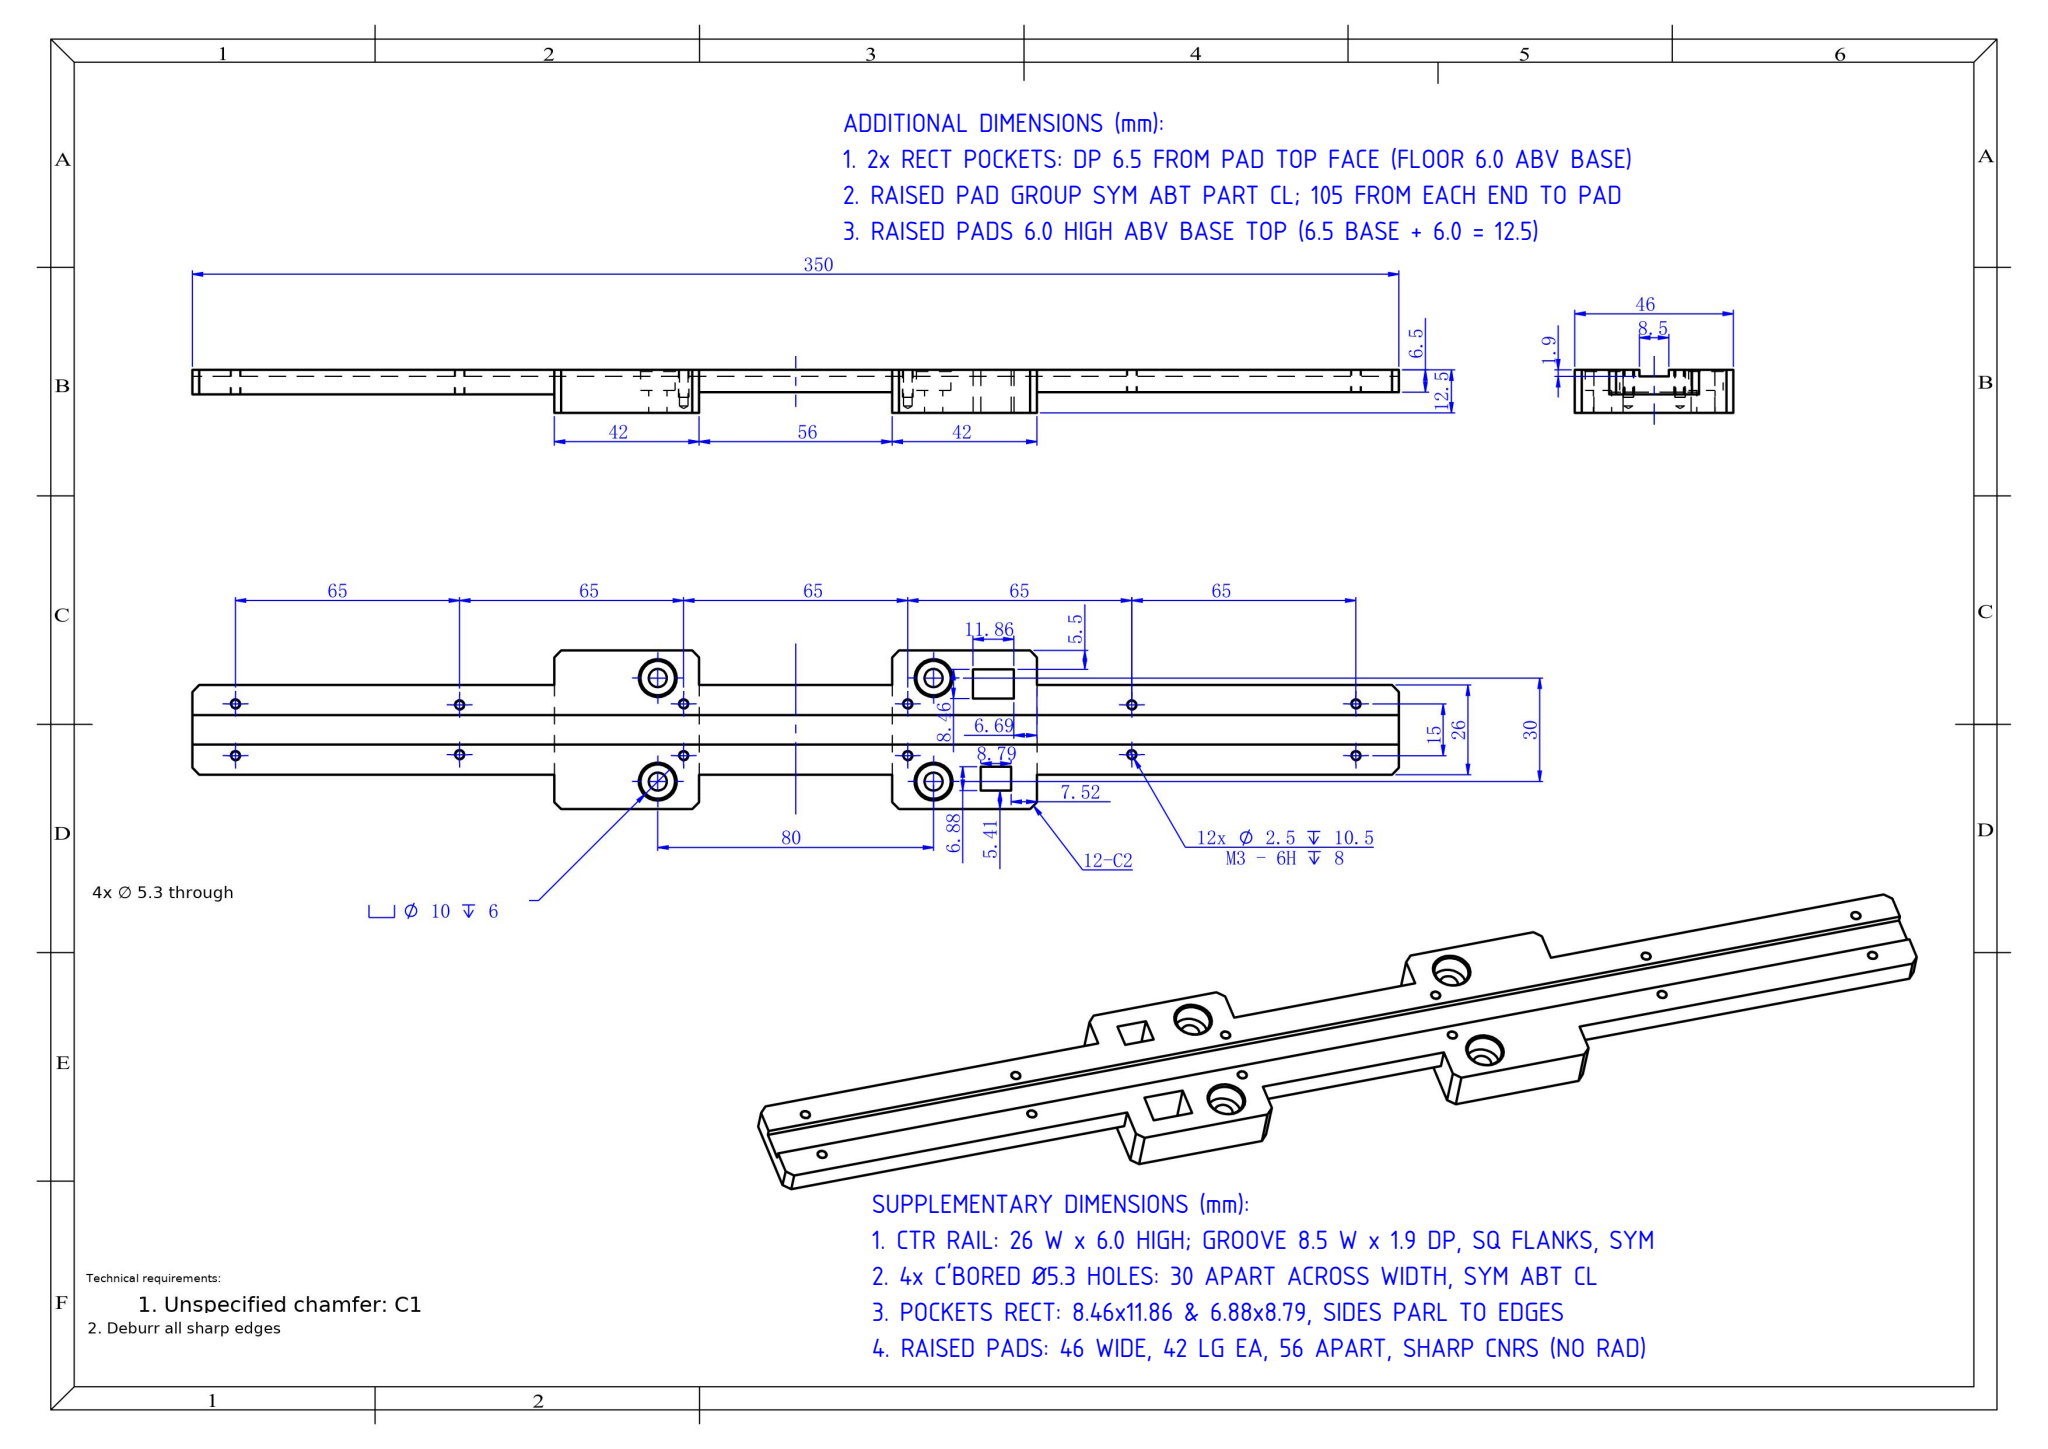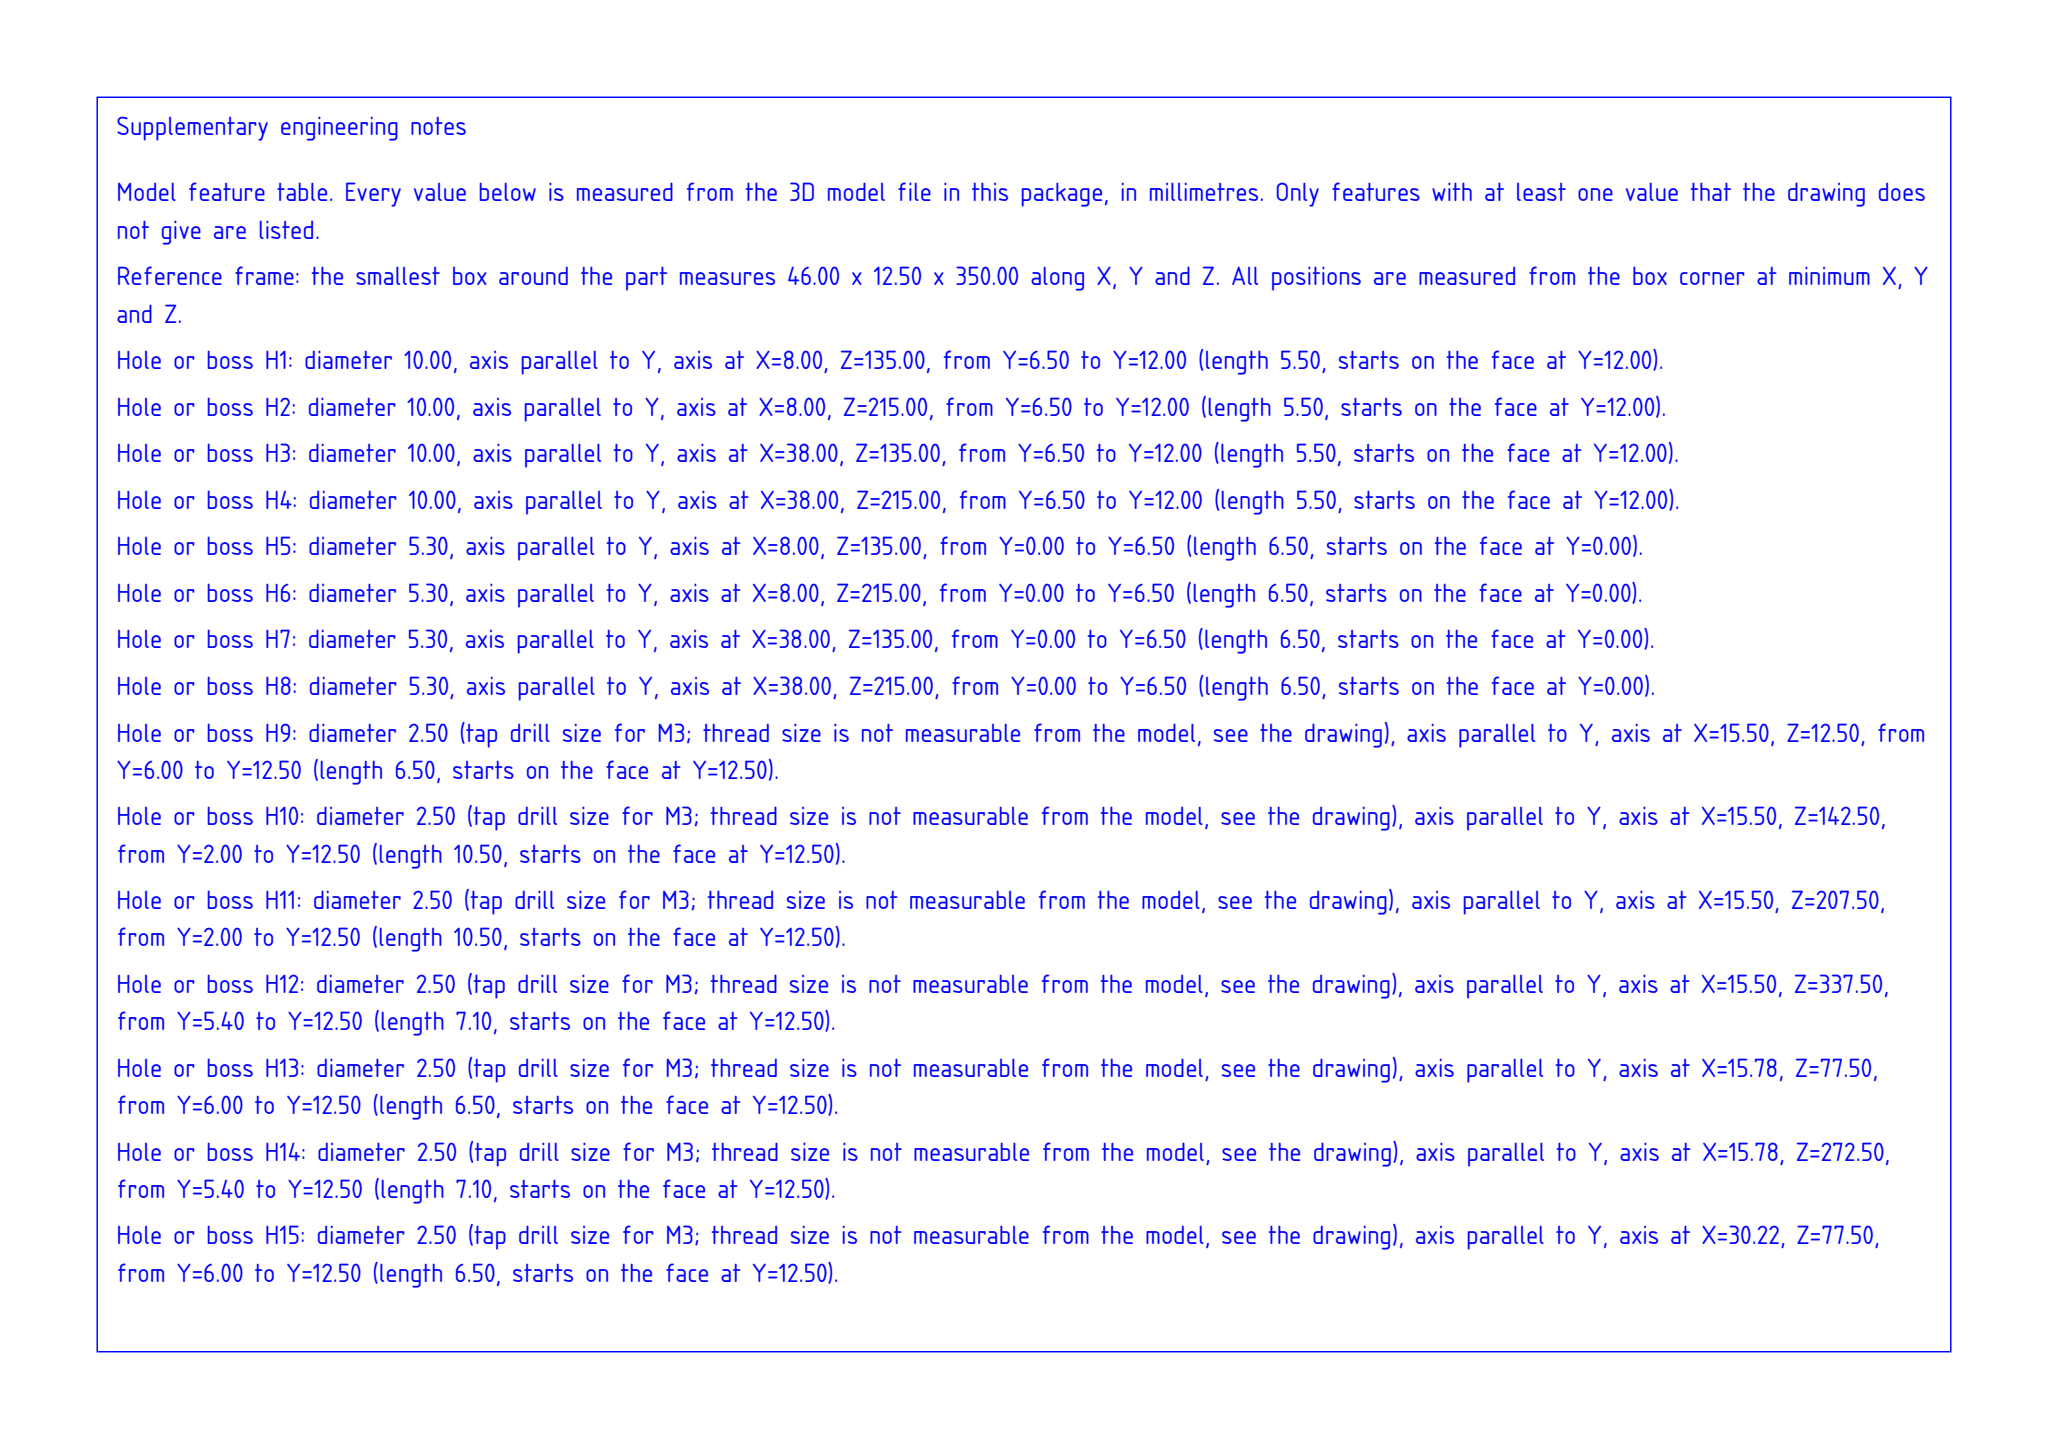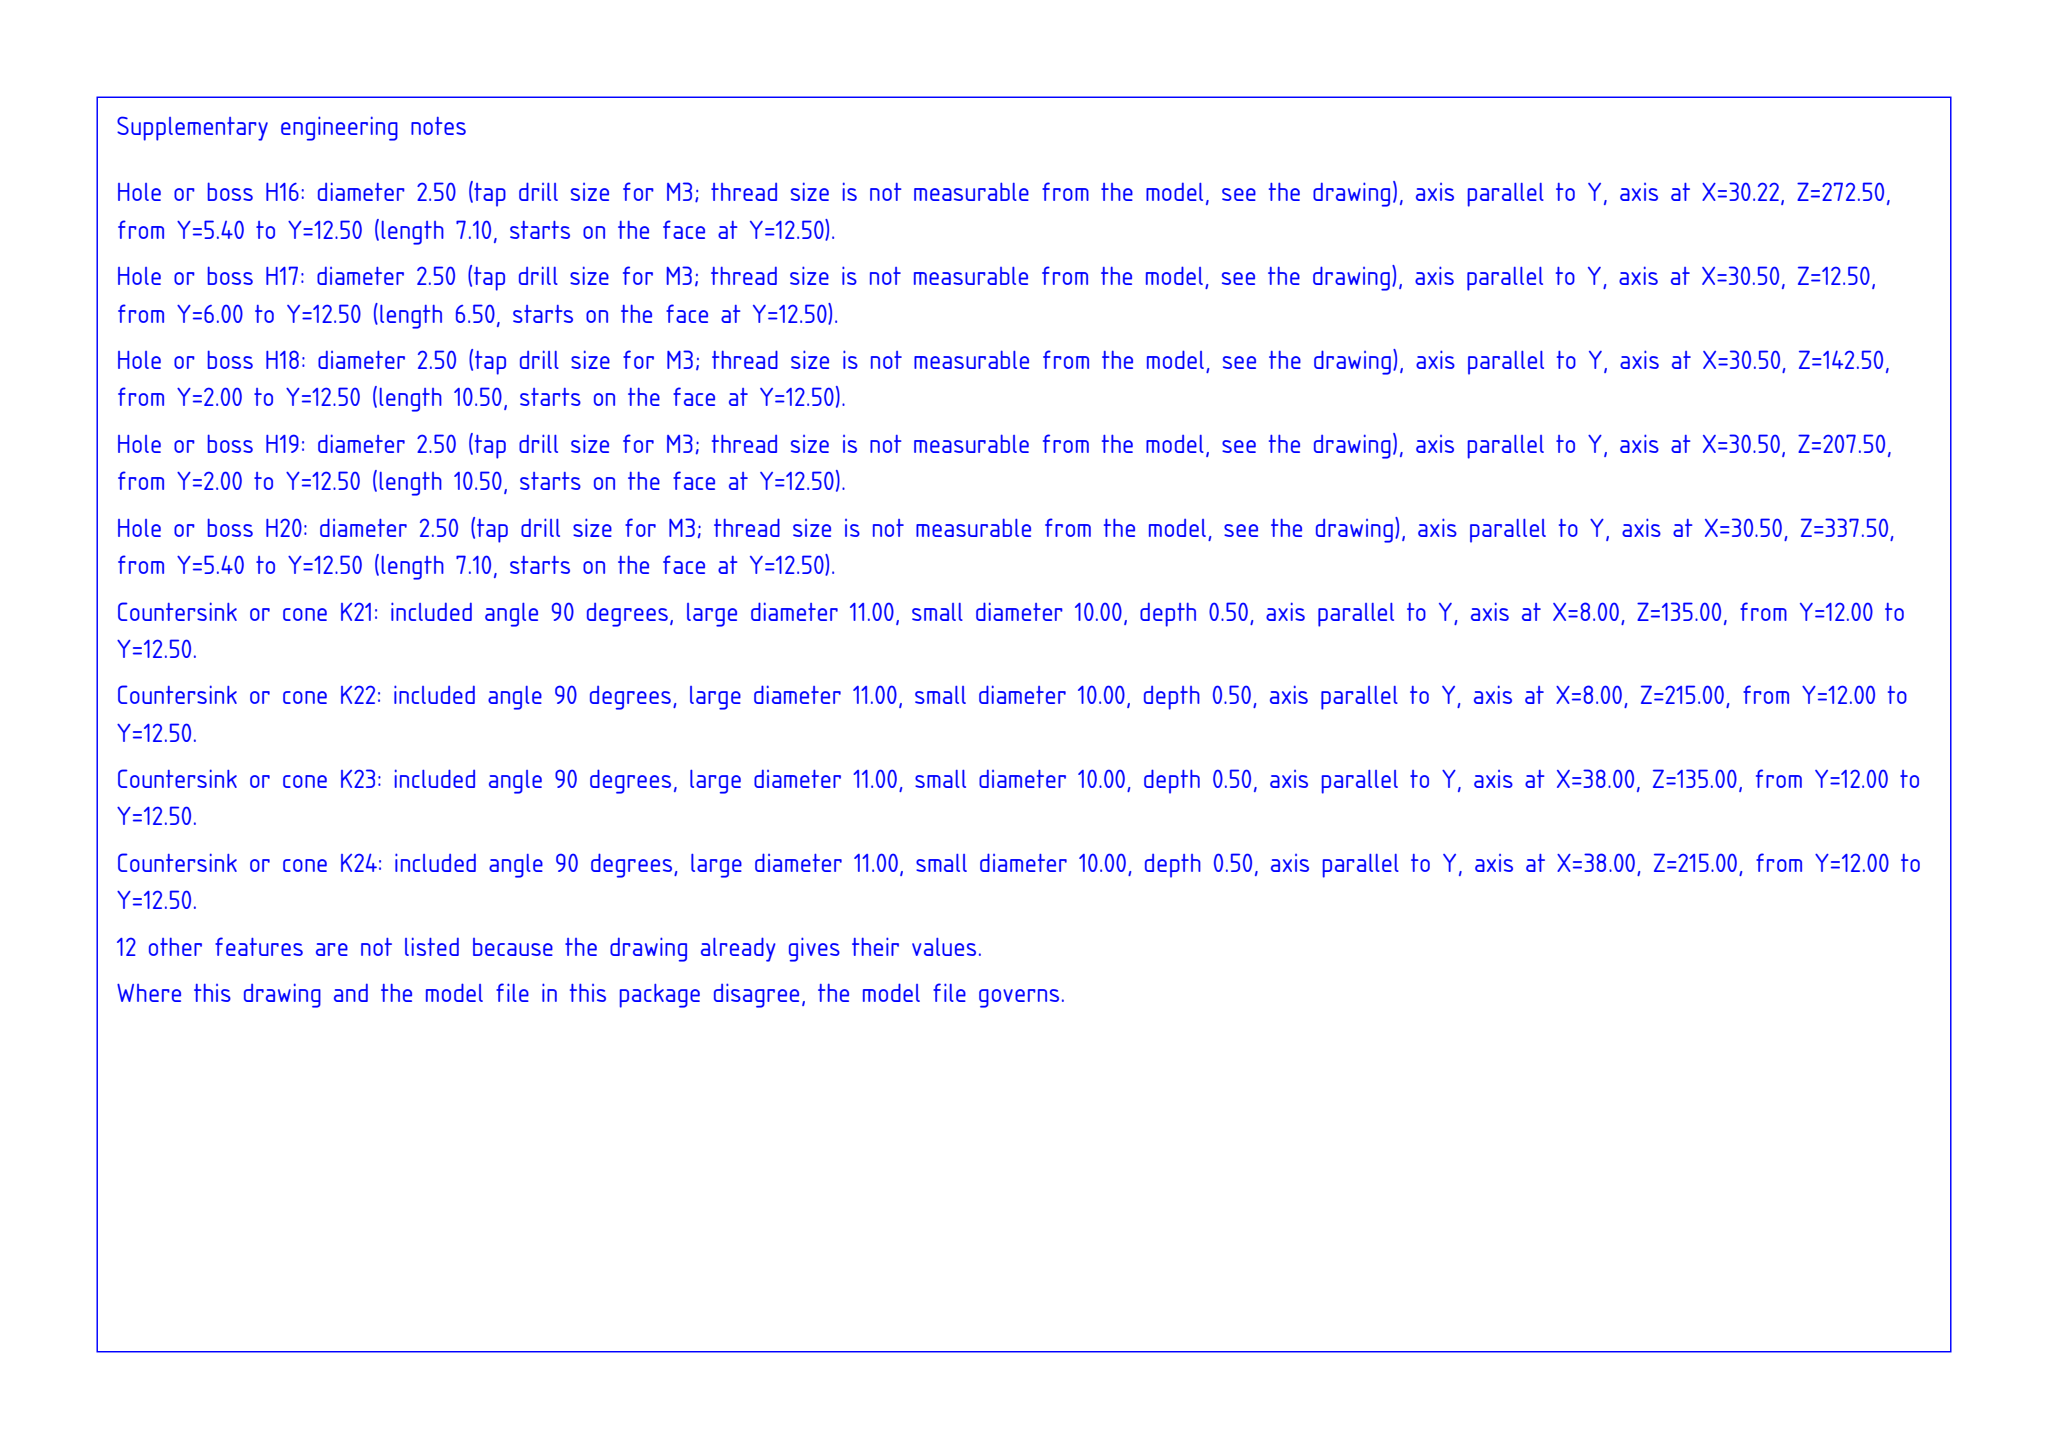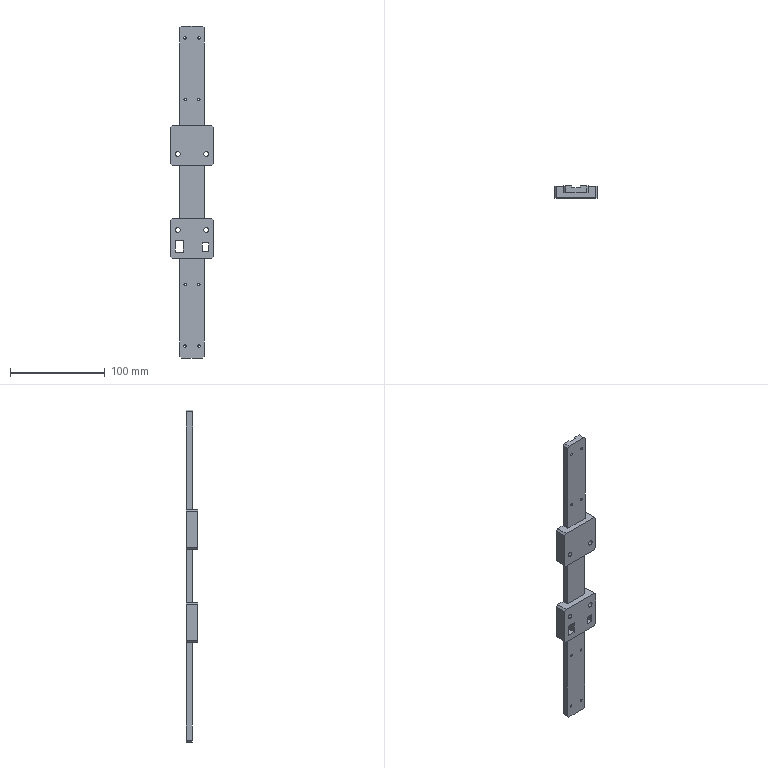Part | SolidWorks | mm | 1 solid | 106 faces | box 46 x 12.5 x 350 mm | volume 84021 mm3 | plane 50 | cylinder 40 | cone 16 | commonest cylinder face diameters 2.5 x24 10 x8 5.3 x8
build123d program:
from build123d import *

# Parameters (mm, degrees)
BOSS_EXTRUDE1_DEPTH                             = 350
M5_HEX_SOCKET_HEAD_CAP_SCREW_CBORE1_D           = 5.3
M5_HEX_SOCKET_HEAD_CAP_SCREW_CBORE1_CBORE_D     = 10
M5_HEX_SOCKET_HEAD_CAP_SCREW_CBORE1_CBORE_DEPTH = 6
CHAMFER1_SIZE                                   = 0.5
SKETCH7_W                                       = 10
SKETCH7_H                                       = 105
CUT_EXTRUDE3_DEPTH                              = 366.908
CHAMFER2_SIZE                                   = 2
SKETCH10_W                                      = 10
SKETCH10_H                                      = 56
CUT_EXTRUDE4_DEPTH                              = 366.908
CHAMFER3_SIZE                                   = 2
SKETCH11_W                                      = 105
SKETCH11_H                                      = 6
SKETCH11_W_2                                    = 56
CUT_EXTRUDE5_DEPTH                              = 355.582
M3_TAPPED_HOLE1_AT_2_COUNT                      = 2
M3_TAPPED_HOLE1_AT_2_PITCH                      = 65.001
M3_TAPPED_HOLE1_AT_3_COUNT                      = 2
M3_TAPPED_HOLE1_AT_3_PITCH                      = 130
M3_TAPPED_HOLE1_AT_4_COUNT                      = 2
M3_TAPPED_HOLE1_AT_4_PITCH                      = 195
M3_TAPPED_HOLE1_AT_5_COUNT                      = 2
M3_TAPPED_HOLE1_AT_5_PITCH                      = 260
M3_TAPPED_HOLE1_AT_6_COUNT                      = 2
M3_TAPPED_HOLE1_AT_6_PITCH                      = 325
SKETCH14_W                                      = 6.885
SKETCH14_H                                      = 8.792
SKETCH14_W_2                                    = 8.461
SKETCH14_H_2                                    = 11.861
CUT_EXTRUDE6_DEPTH                              = 38


with BuildPart() as part:
    # Sketch1 → Boss-Extrude1 (new body)
    with BuildSketch(Plane.XY):
        Polygon((-105.984, 43.956), (-87.234, 43.956), (-87.234, 42.056), (-78.734, 42.056), (-78.734, 43.956), (-59.984, 43.956), (-59.984, 31.456), (-105.984, 31.456), align=None)
    extrude(amount=BOSS_EXTRUDE1_DEPTH)

    # M5 Hex Socket Head Cap Screw CBORE1 (through all)
    with Locations(Plane(origin=(0, 43.956, 0), x_dir=(1, 0, 0), z_dir=(0, 1, 0))):
        with Locations((-67.984, -135), (-67.984, -215), (-97.984, -135), (-97.984, -215)):
            CounterBoreHole(M5_HEX_SOCKET_HEAD_CAP_SCREW_CBORE1_D / 2, M5_HEX_SOCKET_HEAD_CAP_SCREW_CBORE1_CBORE_D / 2, M5_HEX_SOCKET_HEAD_CAP_SCREW_CBORE1_CBORE_DEPTH)

    # Chamfer1
    chamfer1_edges = [part.edges().sort_by_distance(p)[0] for p in [
        (-102.984, 43.956, 215),
        (-102.984, 43.956, 135),
        (-72.984, 43.956, 215),
        (-72.984, 43.956, 135),
    ]]
    chamfer(chamfer1_edges, length=CHAMFER1_SIZE)

    # Sketch7 → Cut-Extrude3 (cut, through all)
    with BuildSketch(Plane(origin=(0, 43.956, 0), x_dir=(1, 0, 0), z_dir=(0, 1, 0))):
        with Locations((-100.984, -52.5)):
            Rectangle(SKETCH7_W, SKETCH7_H)
        with Locations((-100.984, -297.5)):
            Rectangle(SKETCH7_W, SKETCH7_H)
        with Locations((-64.984, -297.5)):
            Rectangle(SKETCH7_W, SKETCH7_H)
        with Locations((-64.984, -52.5)):
            Rectangle(SKETCH7_W, SKETCH7_H)
    extrude(amount=-CUT_EXTRUDE3_DEPTH, mode=Mode.SUBTRACT)

    # Chamfer2
    chamfer2_edges = [part.edges().sort_by_distance(p)[0] for p in [
        (-69.984, 37.706, 0),
        (-59.984, 37.706, 105),
        (-95.984, 37.706, 0),
        (-105.984, 37.706, 105),
        (-105.984, 37.706, 245),
        (-95.984, 37.706, 350),
        (-69.984, 37.706, 350),
        (-59.984, 37.706, 245),
    ]]
    chamfer(chamfer2_edges, length=CHAMFER2_SIZE)

    # Sketch10 → Cut-Extrude4 (cut, through all)
    with BuildSketch(Plane(origin=(0, 43.956, 0), x_dir=(1, 0, 0), z_dir=(0, 1, 0))):
        with Locations((-64.984, -175)):
            Rectangle(SKETCH10_W, SKETCH10_H)
        with Locations((-100.984, -175)):
            Rectangle(SKETCH10_W, SKETCH10_H)
    extrude(amount=-CUT_EXTRUDE4_DEPTH, mode=Mode.SUBTRACT)

    # Chamfer3
    chamfer3_edges = [part.edges().sort_by_distance(p)[0] for p in [
        (-59.984, 37.706, 147),
        (-59.984, 37.706, 203),
        (-105.984, 37.706, 203),
        (-105.984, 37.706, 147),
    ]]
    chamfer(chamfer3_edges, length=CHAMFER3_SIZE)

    # Sketch11 → Cut-Extrude5 (cut, through all)
    with BuildSketch(Plane.ZY.offset(95.984)):
        with Locations((52.5, 34.456)):
            Rectangle(SKETCH11_W, SKETCH11_H)
        with Locations((175, 34.456)):
            Rectangle(SKETCH11_W_2, SKETCH11_H)
        with Locations((297.5, 33.856)):
            Rectangle(SKETCH11_W, SKETCH11_H)
    extrude(amount=-CUT_EXTRUDE5_DEPTH, mode=Mode.SUBTRACT)

    # Sketch13 → M3 Tapped Hole1 (revolve, cut)
    with BuildSketch(Plane(origin=(-90.484, 43.956, 337.5), x_dir=(0, 0, 1), z_dir=(1, 0, 0))):
        Polygon((0, 0), (0, 11.251), (1.25, 10.5), (1.25, 0), align=None)
    m3_tapped_hole1 = revolve(axis=Axis((-90.484, 50.306, 337.5), (0, -1, 0)), mode=Mode.SUBTRACT)

    # M3 Tapped Hole1 at 2: M3 Tapped Hole1 ×2
    with Locations(*[Vector(0.004316, 0, -1) * (i * M3_TAPPED_HOLE1_AT_2_PITCH) for i in range(1, M3_TAPPED_HOLE1_AT_2_COUNT)]):
        add(m3_tapped_hole1, mode=Mode.SUBTRACT)

    # M3 Tapped Hole1 at 3: M3 Tapped Hole1 ×2
    with Locations(*[(0, 0, -i * M3_TAPPED_HOLE1_AT_3_PITCH) for i in range(1, M3_TAPPED_HOLE1_AT_3_COUNT)]):
        add(m3_tapped_hole1, mode=Mode.SUBTRACT)

    # M3 Tapped Hole1 at 4: M3 Tapped Hole1 ×2
    with Locations(*[(0, 0, -i * M3_TAPPED_HOLE1_AT_4_PITCH) for i in range(1, M3_TAPPED_HOLE1_AT_4_COUNT)]):
        add(m3_tapped_hole1, mode=Mode.SUBTRACT)

    # M3 Tapped Hole1 at 5: M3 Tapped Hole1 ×2
    with Locations(*[Vector(0.001079, 0, -1) * (i * M3_TAPPED_HOLE1_AT_5_PITCH) for i in range(1, M3_TAPPED_HOLE1_AT_5_COUNT)]):
        add(m3_tapped_hole1, mode=Mode.SUBTRACT)

    # M3 Tapped Hole1 at 6: M3 Tapped Hole1 ×2
    with Locations(*[(0, 0, -i * M3_TAPPED_HOLE1_AT_6_PITCH) for i in range(1, M3_TAPPED_HOLE1_AT_6_COUNT)]):
        add(m3_tapped_hole1, mode=Mode.SUBTRACT)

    # Mirror1: M3 Tapped Hole1 across plane
    add(m3_tapped_hole1.mirror(Plane(origin=(-82.984, 0, 0), x_dir=(0, 0, 1), z_dir=(1, 0, 0))), mode=Mode.SUBTRACT)

    # Mirror1 copy 1 sketch → Mirror1 copy 1 (revolve, cut)
    with BuildSketch(Plane(origin=(-75.764, 43.956, 272.5), x_dir=(0, 0, 1), z_dir=(-1, 0, 0))):
        Polygon((0, 0), (0, -11.251), (1.25, -10.5), (1.25, 0), align=None)
    revolve(axis=Axis((-75.764, 50.306, 272.5), (0, 1, 0)), mode=Mode.SUBTRACT)

    # Mirror1 copy 2 sketch → Mirror1 copy 2 (revolve, cut)
    with BuildSketch(Plane(origin=(-75.484, 43.956, 207.5), x_dir=(0, 0, 1), z_dir=(-1, 0, 0))):
        Polygon((0, 0), (0, -11.251), (1.25, -10.5), (1.25, 0), align=None)
    revolve(axis=Axis((-75.484, 50.306, 207.5), (0, 1, 0)), mode=Mode.SUBTRACT)

    # Mirror1 copy 3 sketch → Mirror1 copy 3 (revolve, cut)
    with BuildSketch(Plane(origin=(-75.484, 43.956, 142.5), x_dir=(0, 0, 1), z_dir=(-1, 0, 0))):
        Polygon((0, 0), (0, -11.251), (1.25, -10.5), (1.25, 0), align=None)
    revolve(axis=Axis((-75.484, 50.306, 142.5), (0, 1, 0)), mode=Mode.SUBTRACT)

    # Mirror1 copy 4 sketch → Mirror1 copy 4 (revolve, cut)
    with BuildSketch(Plane(origin=(-75.764, 43.956, 77.5), x_dir=(0, 0, 1), z_dir=(-1, 0, 0))):
        Polygon((0, 0), (0, -11.251), (1.25, -10.5), (1.25, 0), align=None)
    revolve(axis=Axis((-75.764, 50.306, 77.5), (0, 1, 0)), mode=Mode.SUBTRACT)

    # Mirror1 copy 5 sketch → Mirror1 copy 5 (revolve, cut)
    with BuildSketch(Plane(origin=(-75.484, 43.956, 12.5), x_dir=(0, 0, 1), z_dir=(-1, 0, 0))):
        Polygon((0, 0), (0, -11.251), (1.25, -10.5), (1.25, 0), align=None)
    revolve(axis=Axis((-75.484, 50.306, 12.5), (0, 1, 0)), mode=Mode.SUBTRACT)

    # Sketch14 → Cut-Extrude6 (cut)
    with BuildSketch(Plane(origin=(0, 43.956, 0), x_dir=(1, 0, 0), z_dir=(0, 1, 0))):
        with Locations((-68.834, -116.915)):
            Rectangle(SKETCH14_W, SKETCH14_H)
        with Locations((-96.248, -117.62)):
            Rectangle(SKETCH14_W_2, SKETCH14_H_2)
    extrude(amount=-CUT_EXTRUDE6_DEPTH, mode=Mode.SUBTRACT)


solid = part.part